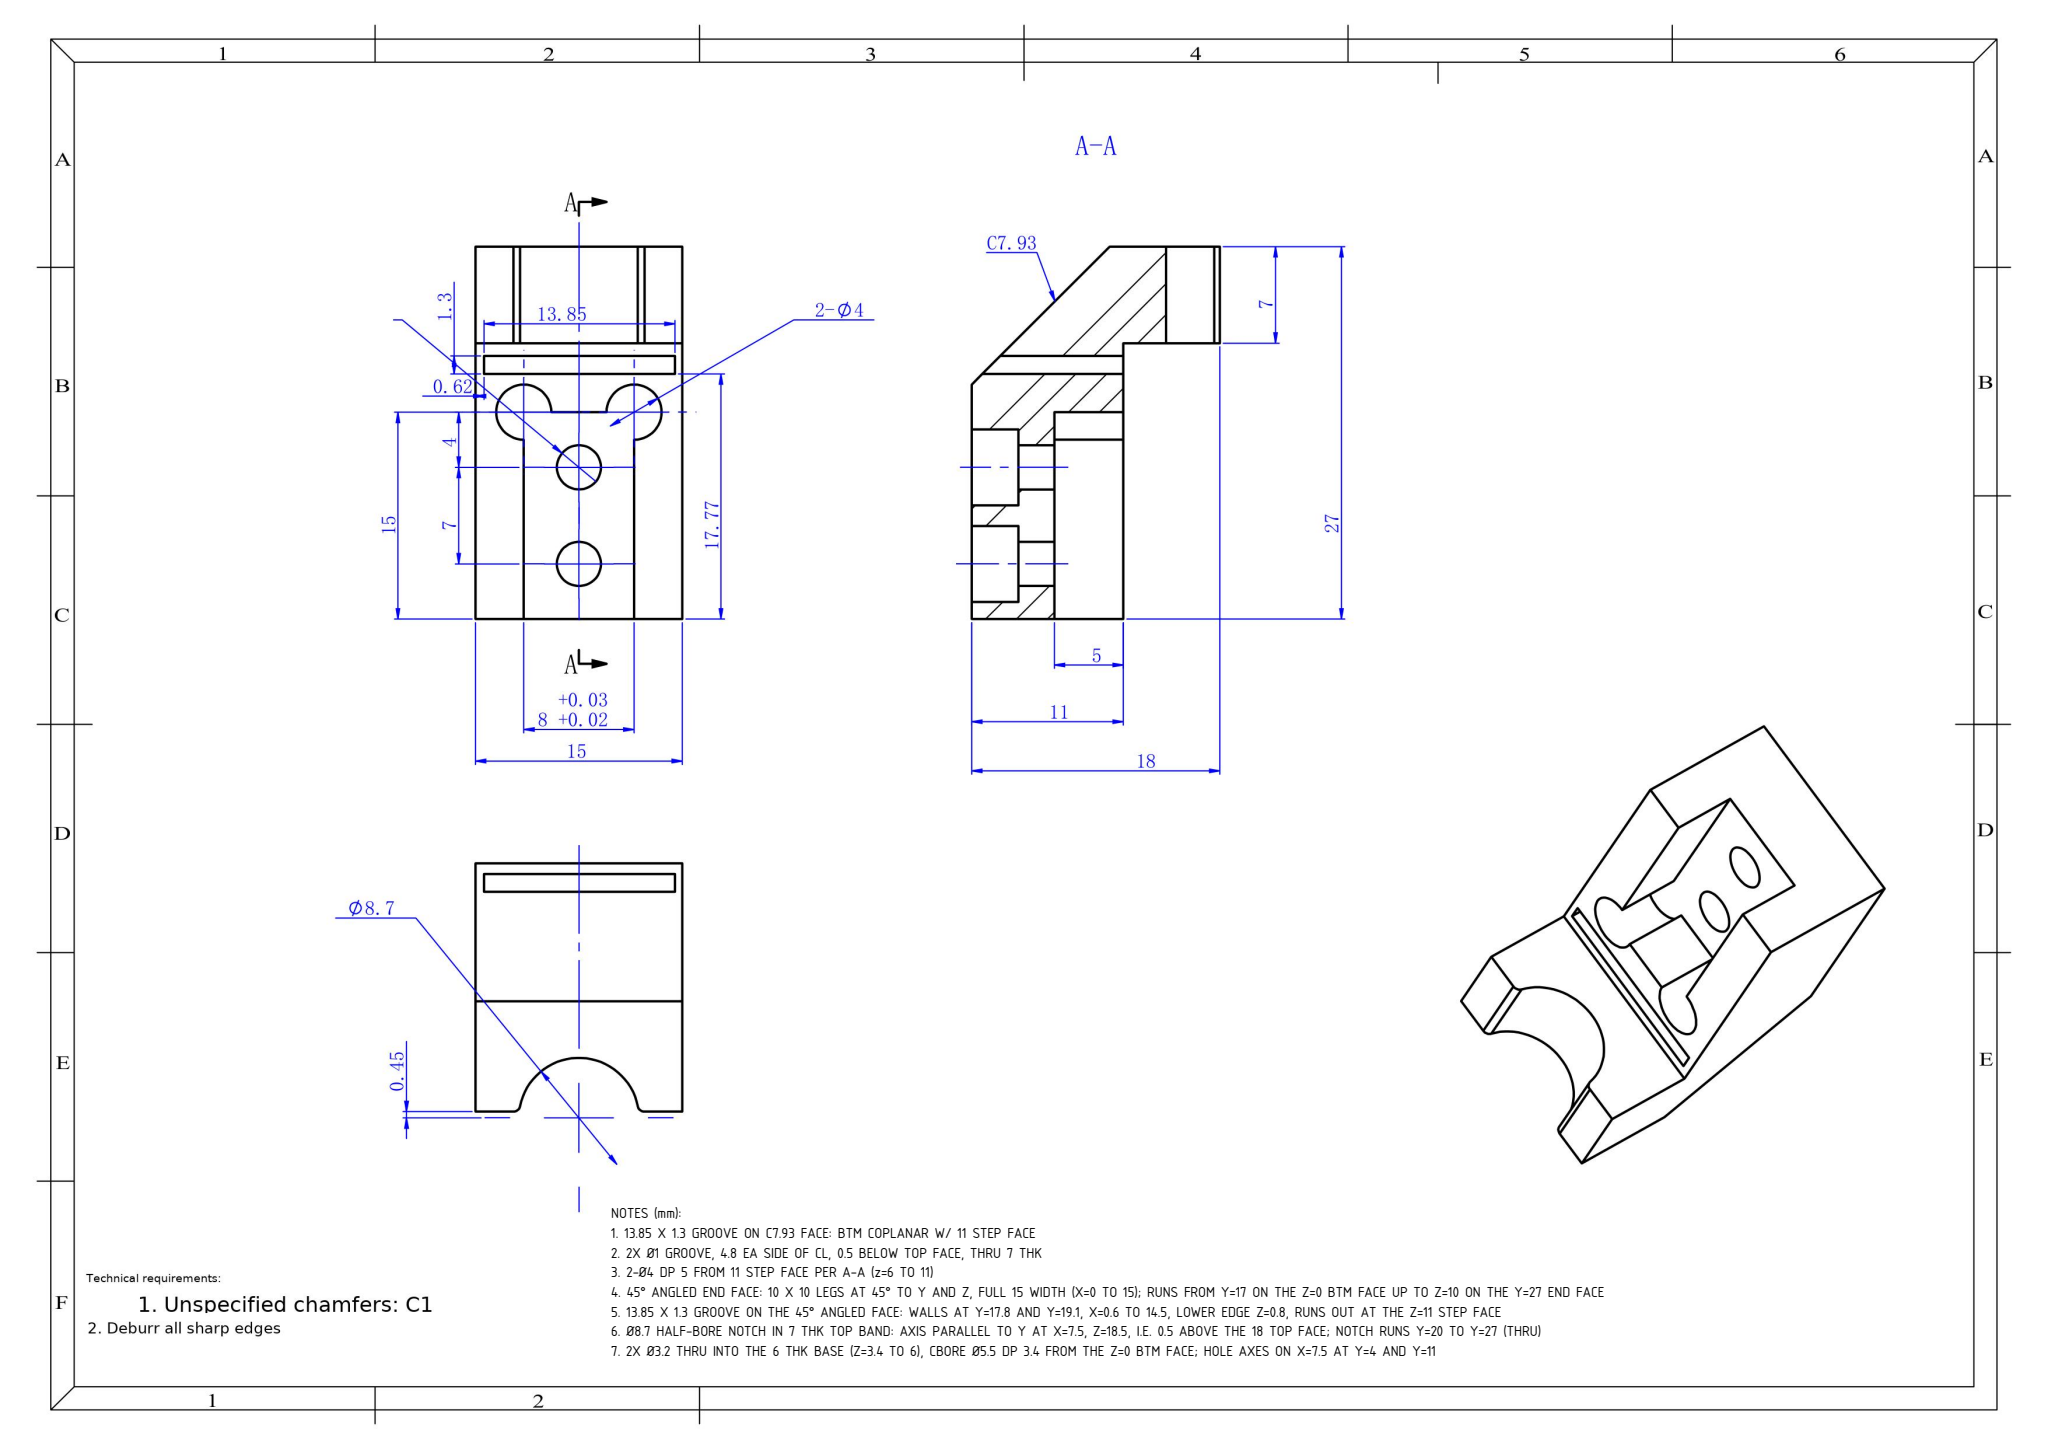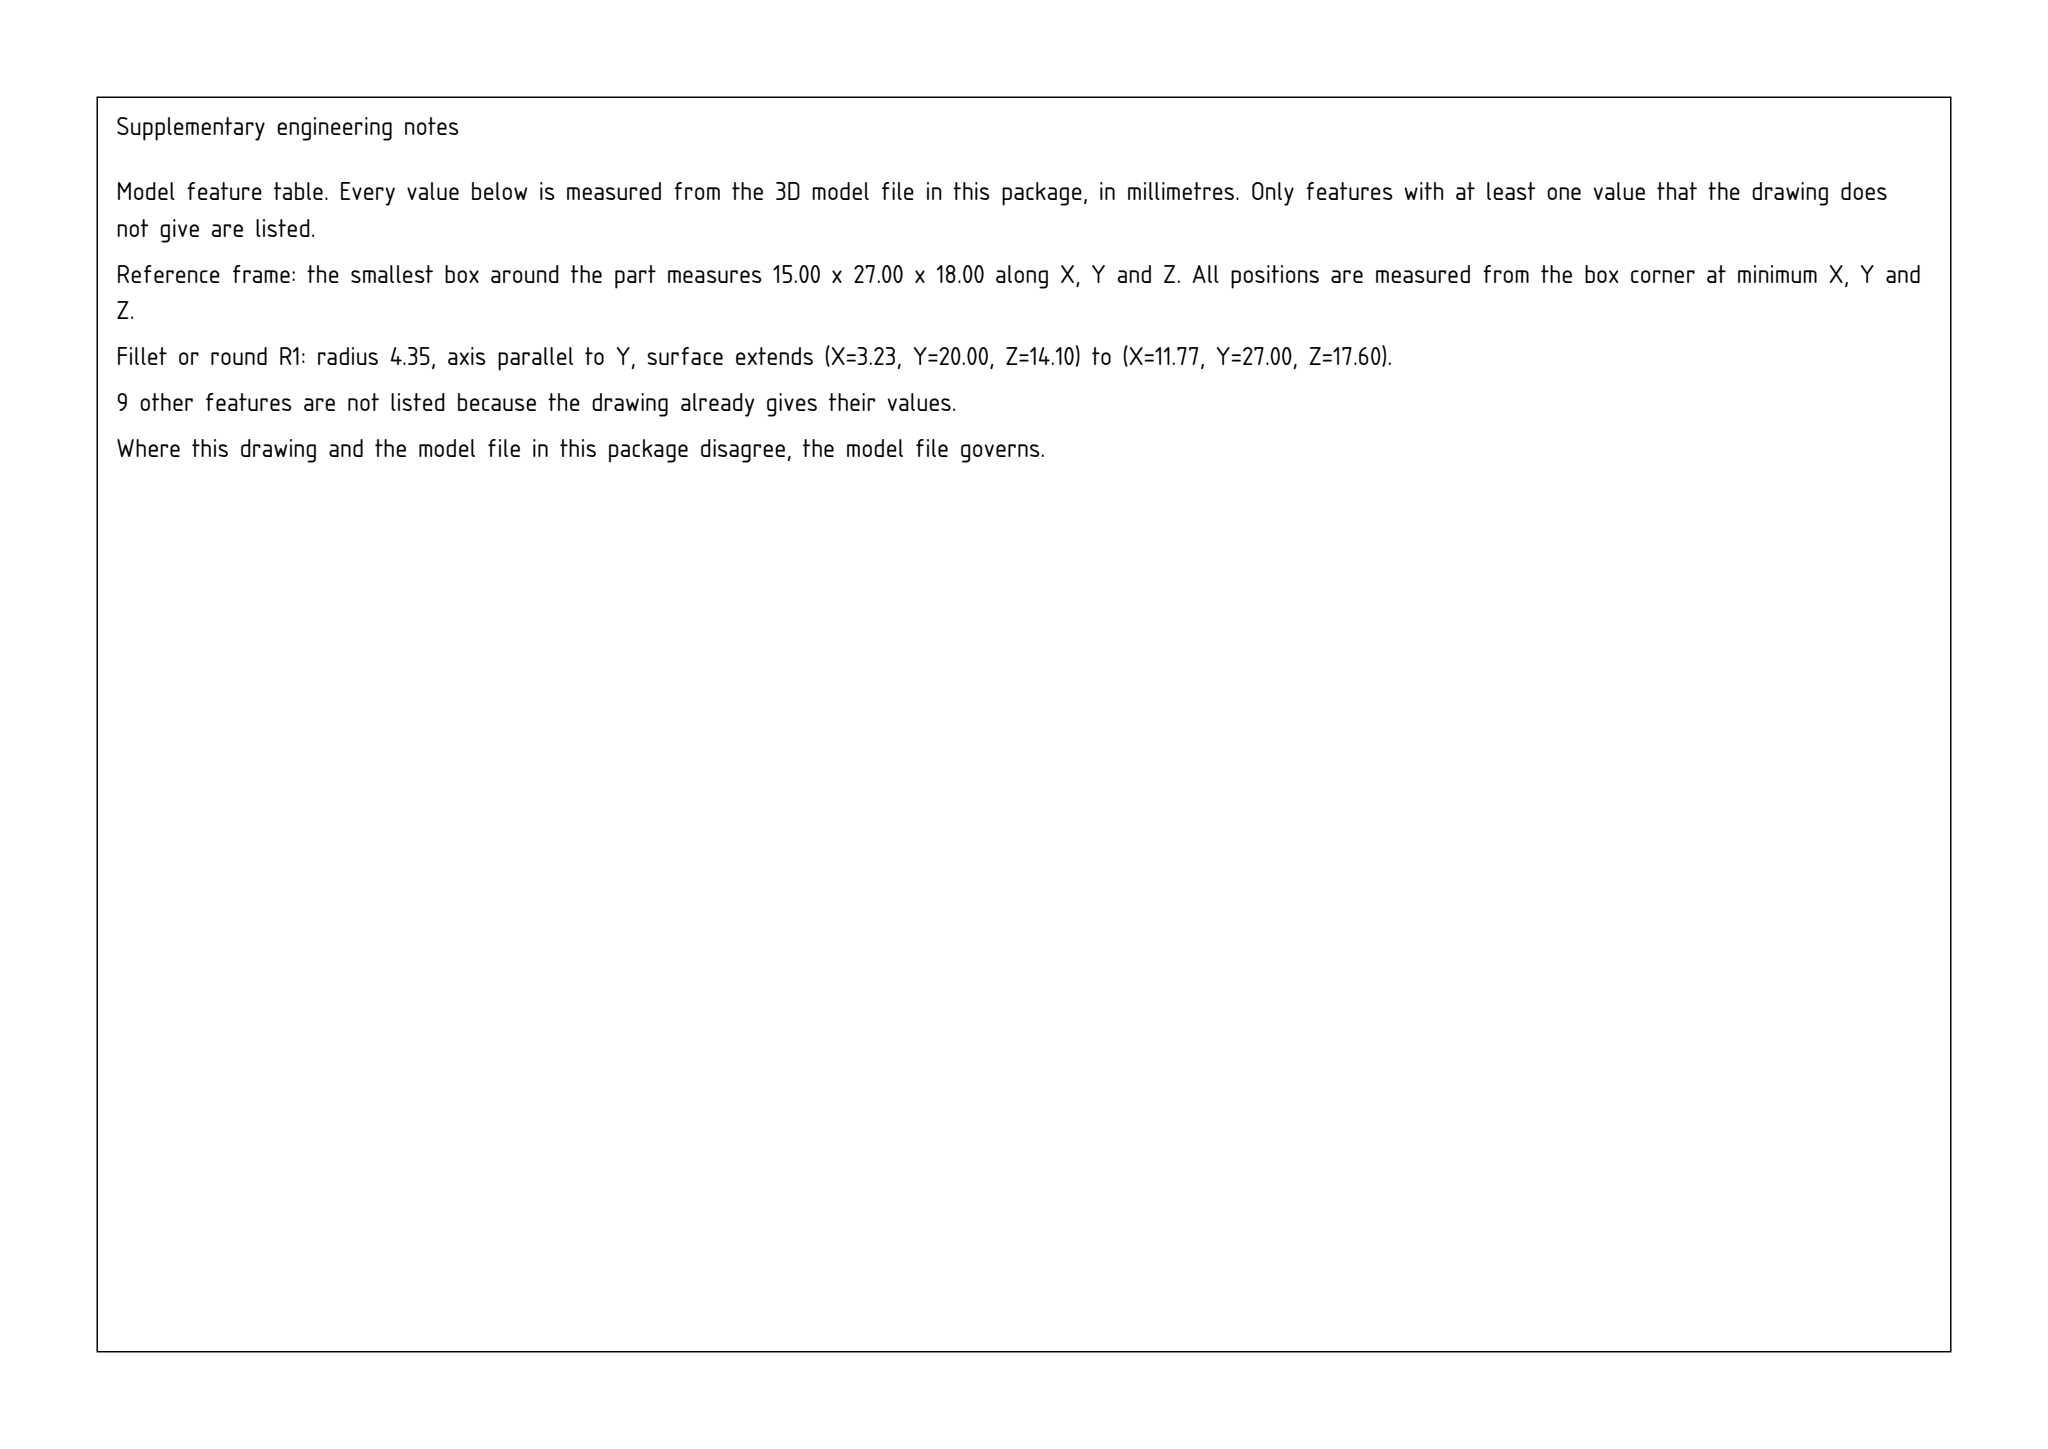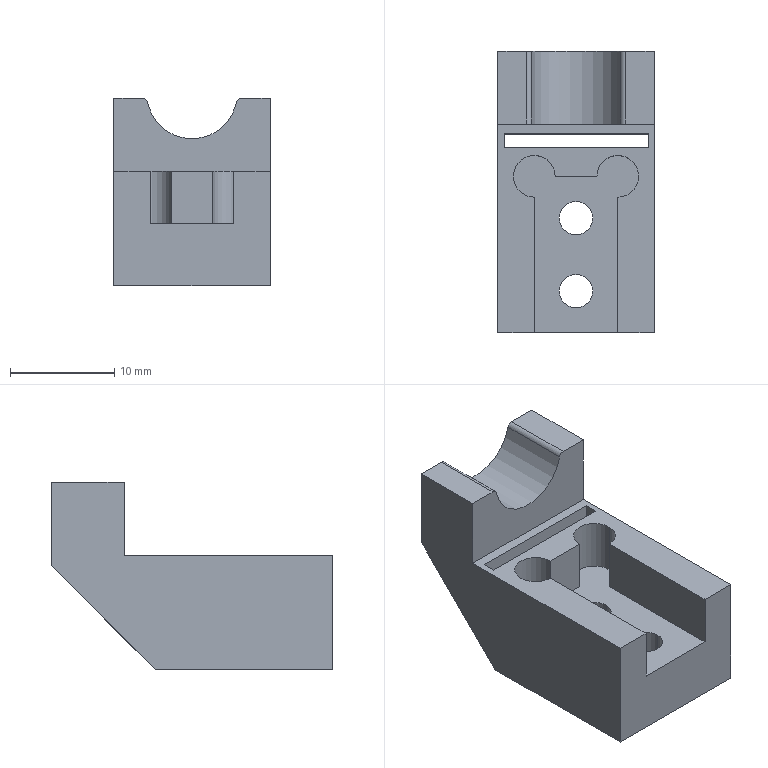Part | SolidWorks | mm | 1 solid | 34 faces | box 15 x 27 x 18 mm | volume 3189 mm3 | plane 20 | cylinder 14 | commonest cylinder face diameters 5.5 x4 3.2 x4 4 x3 1 x2 8.7 x1
Drawing notes:
13.85 X 1.3 GROOVE ON C7.93 FACE: BTM COPLANAR W/ 11 STEP FACE | from the solid: Groove walls y=17.8 (x0.6-14.5, z0.8-11) & y=19.1 (z2.1-11); no inclined btm face - groove btm lies in plane z=11 (same face as the 11 dim in A-A); end walls x=0.6 & x=14.5
2X Ø1 GROOVE, 4.8 EA SIDE OF CL, 0.5 BELOW TOP FACE, THRU 7 THK | from the solid: convex arcs dia 1.0, axis y, at (x=2.7,z=17.5) and (x=12.3,z=17.5), from y=20 to y=27 (7 thk); CL x=7.5, top face z=18
2-Ø4 DP 5 FROM 11 STEP FACE PER A-A (z=6 TO 11) | from the solid: concave arcs dia 4.0, axis z, at (3.5,15) & (11.5,15), from z=6.0 to z=11.0; bounding faces z=6 and z=11
45° ANGLED END FACE: 10 X 10 LEGS AT 45° TO Y AND Z, FULL 15 WIDTH (X=0 TO 15); RUNS FROM Y=17 ON THE Z=0 BTM FACE UP TO Z=10 ON THE Y=27 END FACE | from the solid: inclined_planes: angle_to_xyz_axes [90,45,45], bbox_from [0,17,0], size [15,10,10]; z=0 face extent y 0-17; y=27 face extent z 10-18
13.85 X 1.3 GROOVE ON THE 45° ANGLED FACE: WALLS AT Y=17.8 AND Y=19.1, X=0.6 TO 14.5, LOWER EDGE Z=0.8, RUNS OUT AT THE Z=11 STEP FACE | from the solid: axis_planes y=17.8 (x 0.6-14.5, z 0.8-11), y=19.1 (x 0.6-14.5, z 2.1-11), x=0.6 and x=14.5 (y 17.8-19.1, z 0.8-11)
Ø8.7 HALF-BORE NOTCH IN 7 THK TOP BAND: AXIS PARALLEL TO Y AT X=7.5, Z=18.5, I.E. 0.5 ABOVE THE 18 TOP FACE; NOTCH RUNS Y=20 TO Y=27 (THRU) | from the solid: cylinders: concave arc dia 8.7, axis y, axis_pos [7.5, -, 18.5], from 20 to 27, 157°; z=18 top faces
2X Ø3.2 THRU INTO THE 6 THK BASE (Z=3.4 TO 6), CBORE Ø5.5 DP 3.4 FROM THE Z=0 BTM FACE; HOLE AXES ON X=7.5 AT Y=4 AND Y=11 | from the solid: cylinders: hole/bore dia 3.2 axis z at [7.5,11] and [7.5,4] from 3.4 to 6; hole/bore dia 5.5 axis z at [7.5,11] and [7.5,4] from 0 to 3.4
build123d program:
from build123d import *

# Parameters (mm, degrees)
SKETCH1_W                                       = 15
SKETCH1_H                                       = 27
BOSS_EXTRUDE1_DEPTH                             = 11
SKETCH2_W                                       = 8
SKETCH2_H                                       = 15
CUT_EXTRUDE1_DEPTH                              = 5
M3_HEX_SOCKET_HEAD_CAP_SCREW_CBORE1_D           = 3.2
M3_HEX_SOCKET_HEAD_CAP_SCREW_CBORE1_CBORE_D     = 5.5
M3_HEX_SOCKET_HEAD_CAP_SCREW_CBORE1_CBORE_DEPTH = 3.4
SKETCH5_W                                       = 15
SKETCH5_H                                       = 7
BOSS_EXTRUDE2_DEPTH                             = 7
SKETCH6_R                                       = 4.35
CUT_EXTRUDE3_DEPTH                              = 34.329
FILLET1_R                                       = 0.5
CHAMFER1_SIZE                                   = 10
SKETCH7_R                                       = 2
CUT_EXTRUDE4_DEPTH                              = 5
SKETCH8_W                                       = 13.852
SKETCH8_H                                       = 1.299
CUT_EXTRUDE5_DEPTH                              = 20


with BuildPart() as part:
    # Sketch1 → Boss-Extrude1 (new body)
    with BuildSketch(Plane.XY):
        with Locations((0.1036, 1.036)):
            Rectangle(SKETCH1_W, SKETCH1_H)
    extrude(amount=BOSS_EXTRUDE1_DEPTH)

    # Sketch2 → Cut-Extrude1 (cut)
    with BuildSketch(Plane.XY.offset(11)):
        with Locations((0.1036, -4.964)):
            Rectangle(SKETCH2_W, SKETCH2_H)
    extrude(amount=-CUT_EXTRUDE1_DEPTH, mode=Mode.SUBTRACT)

    # M3 Hex Socket Head Cap Screw CBORE1 (through all)
    with Locations(Plane(origin=(0, 0, 0), x_dir=(-1, 0, 0), z_dir=(0, 0, -1))):
        with Locations((-0.1036, -1.464), (-0.1036, -8.464)):
            CounterBoreHole(M3_HEX_SOCKET_HEAD_CAP_SCREW_CBORE1_D / 2, M3_HEX_SOCKET_HEAD_CAP_SCREW_CBORE1_CBORE_D / 2, M3_HEX_SOCKET_HEAD_CAP_SCREW_CBORE1_CBORE_DEPTH)

    # Sketch5 → Boss-Extrude2 (add)
    with BuildSketch(Plane.XY.offset(11)):
        with Locations((0.1036, 11.036)):
            Rectangle(SKETCH5_W, SKETCH5_H)
    extrude(amount=BOSS_EXTRUDE2_DEPTH)

    # Sketch6 → Cut-Extrude3 (cut, through all)
    with BuildSketch(Plane(origin=(0, 14.536, 0), x_dir=(1, 0, 0), z_dir=(0, 1, 0))):
        with Locations((0.1036, -18.45)):
            Circle(SKETCH6_R)
    extrude(amount=-CUT_EXTRUDE3_DEPTH, mode=Mode.SUBTRACT)

    # Fillet1
    fillet1_edges = [part.edges().sort_by_distance(p)[0] for p in [
        (4.43, 11.036, 18),
        (-4.223, 11.036, 18),
    ]]
    fillet(fillet1_edges, radius=FILLET1_R)

    # Chamfer1
    chamfer1_edges = [part.edges().sort_by_distance(p)[0] for p in [
        (0.1036, 14.536, 0),
    ]]
    chamfer(chamfer1_edges, length=CHAMFER1_SIZE)

    # Sketch7 → Cut-Extrude4 (cut)
    with BuildSketch(Plane.XY.offset(11)):
        with Locations((4.104, 2.536)):
            Circle(SKETCH7_R)
        with Locations((-3.896, 2.536)):
            Circle(SKETCH7_R)
    extrude(amount=-CUT_EXTRUDE4_DEPTH, mode=Mode.SUBTRACT)

    # Sketch8 → Cut-Extrude5 (cut)
    with BuildSketch(Plane.XY.offset(11)):
        with Locations((0.145, 5.957)):
            Rectangle(SKETCH8_W, SKETCH8_H)
    extrude(amount=-CUT_EXTRUDE5_DEPTH, mode=Mode.SUBTRACT)


solid = part.part